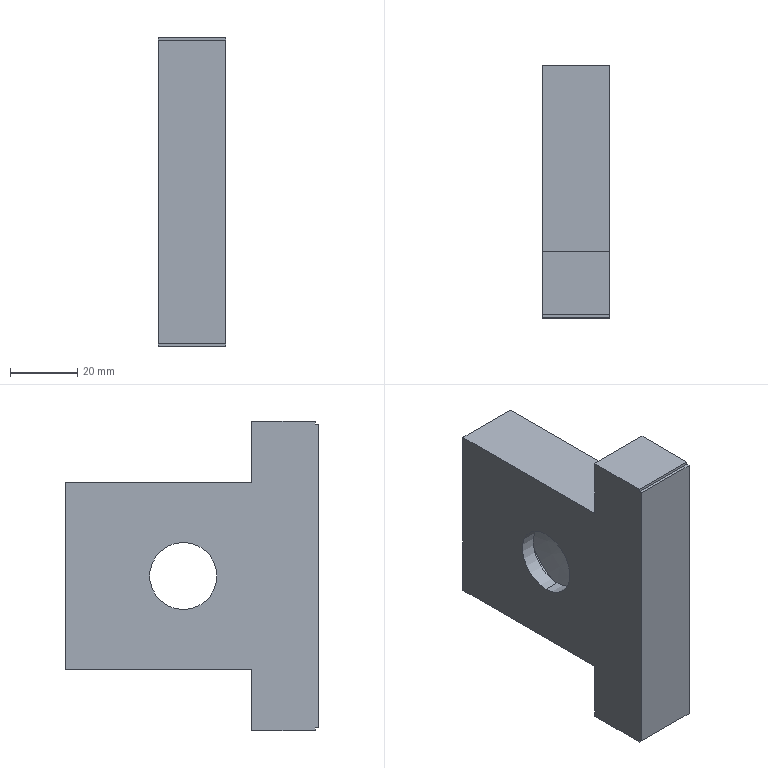Component | SolidWorks | SealingAnvil-1 | 1 solid | 24 faces | box 20 x 75.24 x 92.14 mm | volume 83671 mm3 | plane 14 | cylinder 6 | cone 4 | commonest cylinder face diameters 20 x4 41.575 x2
build123d program:
from build123d import *

# Parameters (mm, degrees)
SKETCH2_R           = 10
BOSS_EXTRUDE1_DEPTH = 20
SKETCH1_W           = 1.15
SKETCH1_H           = 1
CUT_EXTRUDE1_DEPTH  = 108.672


with BuildPart() as part:
    # Sketch2 → Boss-Extrude1 (new body)
    with BuildSketch(Plane.XY):
        Polygon((27.887, 95.24), (-27.887, 95.24), (-27.887, 39.822), (-46.072, 39.822), (-46.072, 20), (46.072, 20), (46.072, 39.822), (27.887, 39.822), align=None)
        with Locations((0, 60.219)):
            Circle(SKETCH2_R, mode=Mode.SUBTRACT)
    extrude(amount=BOSS_EXTRUDE1_DEPTH)

    # Sketch3 → Cut-Revolve1 (revolve, cut)
    with BuildSketch(Plane(origin=(0, 0, 0), x_dir=(0, 0, -1), z_dir=(1, 0, 0)), mode=Mode.PRIVATE) as cut_revolve1_sk:
        Polygon((-12.9, 81.007), (-15.408, 70.219), (-4.592, 70.219), (-7.1, 81.007), align=None)
    revolve(cut_revolve1_sk.sketch.rotate(Axis((0, 60.219, -248), (0, 0, 1)), 90), axis=Axis((0, 60.219, -248), (0, 0, 1)), mode=Mode.SUBTRACT)

    # Sketch1 → Cut-Extrude1 (cut, through all)
    with BuildSketch(Plane.XY.offset(20)):
        with Locations((-45.825, 20.4)):
            Rectangle(SKETCH1_W, SKETCH1_H)
        with Locations((45.825, 20.4)):
            Rectangle(SKETCH1_W, SKETCH1_H)
    extrude(amount=-CUT_EXTRUDE1_DEPTH, mode=Mode.SUBTRACT)


solid = part.part

# Placed as in the assembly
solid = solid.moved(Location((-166, 0, 0), (0, 90, 0)))
STEP:
#1=COLOUR_RGB('',0.7922,0.8196,0.9333);
#2=FILL_AREA_STYLE_COLOUR('',#1);
#3=FILL_AREA_STYLE('',(#2));
#4=SURFACE_STYLE_FILL_AREA(#3);
#5=SURFACE_SIDE_STYLE('',(#4));
#6=SURFACE_STYLE_USAGE(.BOTH.,#5);
#7=PRESENTATION_STYLE_ASSIGNMENT((#6));
#8=CARTESIAN_POINT('',(-6.028,2.371,-0.8184));
#9=VERTEX_POINT('',#8);
#10=CARTESIAN_POINT('',(-6.028,2.371,0.8184));
#11=VERTEX_POINT('',#10);
#12=CARTESIAN_POINT('',(-6.028,2.371,-0.));
#13=DIRECTION('',(-1.,0.,0.));
#14=DIRECTION('',(0.,0.,1.));
#15=AXIS2_PLACEMENT_3D('',#12,#13,#14);
#16=CIRCLE('',#15,0.8184);
#17=EDGE_CURVE('',#9,#11,#16,.T.);
#18=ORIENTED_EDGE('',*,*,#17,.F.);
#19=CARTESIAN_POINT('',(-6.256,2.371,-0.8184));
#20=VERTEX_POINT('',#19);
#21=CARTESIAN_POINT('',(-16.299,2.371,-0.8184));
#22=DIRECTION('',(-1.,0.,0.));
#23=VECTOR('',#22,39.37);
#24=LINE('',#21,#23);
#25=EDGE_CURVE('',#9,#20,#24,.T.);
#26=ORIENTED_EDGE('',*,*,#25,.T.);
#27=CARTESIAN_POINT('',(-6.256,2.371,0.8184));
#28=VERTEX_POINT('',#27);
#29=CARTESIAN_POINT('',(-6.256,2.371,-0.));
#30=DIRECTION('',(-1.,0.,0.));
#31=DIRECTION('',(0.,0.,1.));
#32=AXIS2_PLACEMENT_3D('',#29,#30,#31);
#33=CIRCLE('',#32,0.8184);
#34=EDGE_CURVE('',#20,#28,#33,.T.);
#35=ORIENTED_EDGE('',*,*,#34,.T.);
#36=CARTESIAN_POINT('',(-16.299,2.371,0.8184));
#37=DIRECTION('',(-1.,0.,0.));
#38=VECTOR('',#37,39.37);
#39=LINE('',#36,#38);
#40=EDGE_CURVE('',#11,#28,#39,.T.);
#41=ORIENTED_EDGE('',*,*,#40,.F.);
#42=EDGE_LOOP('',(#18,#26,#35,#41));
#43=FACE_OUTER_BOUND('',#42,.T.);
#44=CARTESIAN_POINT('',(-16.299,2.371,-0.));
#45=DIRECTION('',(-1.,0.,0.));
#46=DIRECTION('',(0.,0.,1.));
#47=AXIS2_PLACEMENT_3D('',#44,#45,#46);
#48=CYLINDRICAL_SURFACE('',#47,0.8184);
#49=ADVANCED_FACE('',(#43),#48,.F.);
#50=CARTESIAN_POINT('',(-6.355,2.371,-0.3937));
#51=VERTEX_POINT('',#50);
#52=CARTESIAN_POINT('',(-6.355,2.371,0.3937));
#53=VERTEX_POINT('',#52);
#54=CARTESIAN_POINT('',(-6.355,2.371,-0.));
#55=DIRECTION('',(-1.,0.,0.));
#56=DIRECTION('',(0.,0.,1.));
#57=AXIS2_PLACEMENT_3D('',#54,#55,#56);
#58=CIRCLE('',#57,0.3937);
#59=EDGE_CURVE('',#51,#53,#58,.T.);
#60=ORIENTED_EDGE('',*,*,#59,.T.);
#61=CARTESIAN_POINT('',(-6.355,2.371,0.3937));
#62=DIRECTION('',(0.2264,0.,0.974));
#63=VECTOR('',#62,39.37);
#64=LINE('',#61,#63);
#65=EDGE_CURVE('',#53,#28,#64,.T.);
#66=ORIENTED_EDGE('',*,*,#65,.T.);
#67=ORIENTED_EDGE('',*,*,#34,.F.);
#68=CARTESIAN_POINT('',(-6.355,2.371,-0.3937));
#69=DIRECTION('',(0.2264,0.,-0.974));
#70=VECTOR('',#69,39.37);
#71=LINE('',#68,#70);
#72=EDGE_CURVE('',#51,#20,#71,.T.);
#73=ORIENTED_EDGE('',*,*,#72,.F.);
#74=EDGE_LOOP('',(#60,#66,#67,#73));
#75=FACE_OUTER_BOUND('',#74,.T.);
#76=CARTESIAN_POINT('',(-6.355,2.371,-0.));
#77=DIRECTION('',(1.,0.,0.));
#78=DIRECTION('',(0.,0.,-1.));
#79=AXIS2_PLACEMENT_3D('',#76,#77,#78);
#80=CONICAL_SURFACE('',#79,0.3937,1.342);
#81=ADVANCED_FACE('',(#75),#80,.F.);
#82=CARTESIAN_POINT('',(-5.929,2.371,-0.3937));
#83=VERTEX_POINT('',#82);
#84=CARTESIAN_POINT('',(-5.929,2.371,0.3937));
#85=VERTEX_POINT('',#84);
#86=CARTESIAN_POINT('',(-5.929,2.371,-0.));
#87=DIRECTION('',(-1.,0.,0.));
#88=DIRECTION('',(0.,0.,1.));
#89=AXIS2_PLACEMENT_3D('',#86,#87,#88);
#90=CIRCLE('',#89,0.3937);
#91=EDGE_CURVE('',#83,#85,#90,.T.);
#92=ORIENTED_EDGE('',*,*,#91,.F.);
#93=CARTESIAN_POINT('',(-5.929,2.371,-0.3937));
#94=DIRECTION('',(-0.2264,0.,-0.974));
#95=VECTOR('',#94,39.37);
#96=LINE('',#93,#95);
#97=EDGE_CURVE('',#83,#9,#96,.T.);
#98=ORIENTED_EDGE('',*,*,#97,.T.);
#99=ORIENTED_EDGE('',*,*,#17,.T.);
#100=CARTESIAN_POINT('',(-5.929,2.371,0.3937));
#101=DIRECTION('',(-0.2264,0.,0.974));
#102=VECTOR('',#101,39.37);
#103=LINE('',#100,#102);
#104=EDGE_CURVE('',#85,#11,#103,.T.);
#105=ORIENTED_EDGE('',*,*,#104,.F.);
#106=EDGE_LOOP('',(#92,#98,#99,#105));
#107=FACE_OUTER_BOUND('',#106,.T.);
#108=CARTESIAN_POINT('',(-5.929,2.371,-0.));
#109=DIRECTION('',(-1.,0.,0.));
#110=DIRECTION('',(0.,0.,1.));
#111=AXIS2_PLACEMENT_3D('',#108,#109,#110);
#112=CONICAL_SURFACE('',#111,0.3937,1.342);
#113=ADVANCED_FACE('',(#107),#112,.F.);
#114=ORIENTED_EDGE('',*,*,#59,.F.);
#115=CARTESIAN_POINT('',(-6.535,2.371,-0.3937));
#116=VERTEX_POINT('',#115);
#117=CARTESIAN_POINT('',(-5.748,2.371,-0.3937));
#118=DIRECTION('',(-1.,0.,0.));
#119=VECTOR('',#118,39.37);
#120=LINE('',#117,#119);
#121=EDGE_CURVE('',#51,#116,#120,.T.);
#122=ORIENTED_EDGE('',*,*,#121,.T.);
#123=CARTESIAN_POINT('',(-6.535,2.371,0.3937));
#124=VERTEX_POINT('',#123);
#125=CARTESIAN_POINT('',(-6.535,2.371,-0.));
#126=DIRECTION('',(1.,0.,0.));
#127=DIRECTION('',(0.,0.,-1.));
#128=AXIS2_PLACEMENT_3D('',#125,#126,#127);
#129=CIRCLE('',#128,0.3937);
#130=EDGE_CURVE('',#124,#116,#129,.T.);
#131=ORIENTED_EDGE('',*,*,#130,.F.);
#132=CARTESIAN_POINT('',(-5.748,2.371,0.3937));
#133=DIRECTION('',(-1.,0.,0.));
#134=VECTOR('',#133,39.37);
#135=LINE('',#132,#134);
#136=EDGE_CURVE('',#53,#124,#135,.T.);
#137=ORIENTED_EDGE('',*,*,#136,.F.);
#138=EDGE_LOOP('',(#114,#122,#131,#137));
#139=FACE_OUTER_BOUND('',#138,.T.);
#140=CARTESIAN_POINT('',(-5.748,2.371,-0.));
#141=DIRECTION('',(-1.,0.,0.));
#142=DIRECTION('',(0.,0.,1.));
#143=AXIS2_PLACEMENT_3D('',#140,#141,#142);
#144=CYLINDRICAL_SURFACE('',#143,0.3937);
#145=ADVANCED_FACE('',(#139),#144,.F.);
#146=CARTESIAN_POINT('',(-5.748,2.371,0.3937));
#147=VERTEX_POINT('',#146);
#148=CARTESIAN_POINT('',(-5.748,2.371,-0.3937));
#149=VERTEX_POINT('',#148);
#150=CARTESIAN_POINT('',(-5.748,2.371,-0.));
#151=DIRECTION('',(1.,0.,0.));
#152=DIRECTION('',(0.,0.,-1.));
#153=AXIS2_PLACEMENT_3D('',#150,#151,#152);
#154=CIRCLE('',#153,0.3937);
#155=EDGE_CURVE('',#147,#149,#154,.T.);
#156=ORIENTED_EDGE('',*,*,#155,.T.);
#157=CARTESIAN_POINT('',(-5.748,2.371,-0.3937));
#158=DIRECTION('',(-1.,0.,0.));
#159=VECTOR('',#158,39.37);
#160=LINE('',#157,#159);
#161=EDGE_CURVE('',#149,#83,#160,.T.);
#162=ORIENTED_EDGE('',*,*,#161,.T.);
#163=ORIENTED_EDGE('',*,*,#91,.T.);
#164=CARTESIAN_POINT('',(-5.748,2.371,0.3937));
#165=DIRECTION('',(-1.,0.,0.));
#166=VECTOR('',#165,39.37);
#167=LINE('',#164,#166);
#168=EDGE_CURVE('',#147,#85,#167,.T.);
#169=ORIENTED_EDGE('',*,*,#168,.F.);
#170=EDGE_LOOP('',(#156,#162,#163,#169));
#171=FACE_OUTER_BOUND('',#170,.T.);
#172=CARTESIAN_POINT('',(-5.748,2.371,-0.));
#173=DIRECTION('',(-1.,0.,0.));
#174=DIRECTION('',(0.,0.,1.));
#175=AXIS2_PLACEMENT_3D('',#172,#173,#174);
#176=CYLINDRICAL_SURFACE('',#175,0.3937);
#177=ADVANCED_FACE('',(#171),#176,.F.);
#178=ORIENTED_EDGE('',*,*,#161,.F.);
#179=CARTESIAN_POINT('',(-5.748,2.371,-0.));
#180=DIRECTION('',(1.,0.,0.));
#181=DIRECTION('',(0.,0.,-1.));
#182=AXIS2_PLACEMENT_3D('',#179,#180,#181);
#183=CIRCLE('',#182,0.3937);
#184=EDGE_CURVE('',#149,#147,#183,.T.);
#185=ORIENTED_EDGE('',*,*,#184,.T.);
#186=ORIENTED_EDGE('',*,*,#168,.T.);
#187=CARTESIAN_POINT('',(-5.929,2.371,-0.));
#188=DIRECTION('',(-1.,0.,0.));
#189=DIRECTION('',(0.,0.,1.));
#190=AXIS2_PLACEMENT_3D('',#187,#188,#189);
#191=CIRCLE('',#190,0.3937);
#192=EDGE_CURVE('',#85,#83,#191,.T.);
#193=ORIENTED_EDGE('',*,*,#192,.T.);
#194=EDGE_LOOP('',(#178,#185,#186,#193));
#195=FACE_OUTER_BOUND('',#194,.T.);
#196=CARTESIAN_POINT('',(-5.748,2.371,-0.));
#197=DIRECTION('',(-1.,0.,0.));
#198=DIRECTION('',(0.,0.,1.));
#199=AXIS2_PLACEMENT_3D('',#196,#197,#198);
#200=CYLINDRICAL_SURFACE('',#199,0.3937);
#201=ADVANCED_FACE('',(#195),#200,.F.);
#202=CARTESIAN_POINT('',(-5.748,0.7874,1.781));
#203=VERTEX_POINT('',#202);
#204=CARTESIAN_POINT('',(-5.748,0.8228,1.781));
#205=VERTEX_POINT('',#204);
#206=CARTESIAN_POINT('',(-5.748,0.7835,1.781));
#207=DIRECTION('',(0.,1.,0.));
#208=VECTOR('',#207,39.37);
#209=LINE('',#206,#208);
#210=EDGE_CURVE('',#203,#205,#209,.T.);
#211=ORIENTED_EDGE('',*,*,#210,.F.);
#212=CARTESIAN_POINT('',(-5.748,0.7874,-1.781));
#213=VERTEX_POINT('',#212);
#214=CARTESIAN_POINT('',(-5.748,0.7874,1.814));
#215=DIRECTION('',(0.,0.,-1.));
#216=VECTOR('',#215,39.37);
#217=LINE('',#214,#216);
#218=EDGE_CURVE('',#203,#213,#217,.T.);
#219=ORIENTED_EDGE('',*,*,#218,.T.);
#220=CARTESIAN_POINT('',(-5.748,0.8228,-1.781));
#221=VERTEX_POINT('',#220);
#222=CARTESIAN_POINT('',(-5.748,0.7835,-1.781));
#223=DIRECTION('',(0.,-1.,0.));
#224=VECTOR('',#223,39.37);
#225=LINE('',#222,#224);
#226=EDGE_CURVE('',#221,#213,#225,.T.);
#227=ORIENTED_EDGE('',*,*,#226,.F.);
#228=CARTESIAN_POINT('',(-5.748,0.8228,-1.814));
#229=VERTEX_POINT('',#228);
#230=CARTESIAN_POINT('',(-5.748,0.8228,-1.827));
#231=DIRECTION('',(0.,0.,1.));
#232=VECTOR('',#231,39.37);
#233=LINE('',#230,#232);
#234=EDGE_CURVE('',#229,#221,#233,.T.);
#235=ORIENTED_EDGE('',*,*,#234,.F.);
#236=CARTESIAN_POINT('',(-5.748,1.568,-1.814));
#237=VERTEX_POINT('',#236);
#238=CARTESIAN_POINT('',(-5.748,0.7874,-1.814));
#239=DIRECTION('',(0.,1.,0.));
#240=VECTOR('',#239,39.37);
#241=LINE('',#238,#240);
#242=EDGE_CURVE('',#229,#237,#241,.T.);
#243=ORIENTED_EDGE('',*,*,#242,.T.);
#244=CARTESIAN_POINT('',(-5.748,1.568,-1.098));
#245=VERTEX_POINT('',#244);
#246=CARTESIAN_POINT('',(-5.748,1.568,-1.814));
#247=DIRECTION('',(0.,0.,1.));
#248=VECTOR('',#247,39.37);
#249=LINE('',#246,#248);
#250=EDGE_CURVE('',#237,#245,#249,.T.);
#251=ORIENTED_EDGE('',*,*,#250,.T.);
#252=CARTESIAN_POINT('',(-5.748,3.75,-1.098));
#253=VERTEX_POINT('',#252);
#254=CARTESIAN_POINT('',(-5.748,1.568,-1.098));
#255=DIRECTION('',(0.,1.,0.));
#256=VECTOR('',#255,39.37);
#257=LINE('',#254,#256);
#258=EDGE_CURVE('',#245,#253,#257,.T.);
#259=ORIENTED_EDGE('',*,*,#258,.T.);
#260=CARTESIAN_POINT('',(-5.748,3.75,1.098));
#261=VERTEX_POINT('',#260);
#262=CARTESIAN_POINT('',(-5.748,3.75,-1.098));
#263=DIRECTION('',(0.,0.,1.));
#264=VECTOR('',#263,39.37);
#265=LINE('',#262,#264);
#266=EDGE_CURVE('',#253,#261,#265,.T.);
#267=ORIENTED_EDGE('',*,*,#266,.T.);
#268=CARTESIAN_POINT('',(-5.748,1.568,1.098));
#269=VERTEX_POINT('',#268);
#270=CARTESIAN_POINT('',(-5.748,3.75,1.098));
#271=DIRECTION('',(0.,-1.,0.));
#272=VECTOR('',#271,39.37);
#273=LINE('',#270,#272);
#274=EDGE_CURVE('',#261,#269,#273,.T.);
#275=ORIENTED_EDGE('',*,*,#274,.T.);
#276=CARTESIAN_POINT('',(-5.748,1.568,1.814));
#277=VERTEX_POINT('',#276);
#278=CARTESIAN_POINT('',(-5.748,1.568,1.098));
#279=DIRECTION('',(0.,-0.,1.));
#280=VECTOR('',#279,39.37);
#281=LINE('',#278,#280);
#282=EDGE_CURVE('',#269,#277,#281,.T.);
#283=ORIENTED_EDGE('',*,*,#282,.T.);
#284=CARTESIAN_POINT('',(-5.748,0.8228,1.814));
#285=VERTEX_POINT('',#284);
#286=CARTESIAN_POINT('',(-5.748,1.568,1.814));
#287=DIRECTION('',(0.,-1.,-0.));
#288=VECTOR('',#287,39.37);
#289=LINE('',#286,#288);
#290=EDGE_CURVE('',#277,#285,#289,.T.);
#291=ORIENTED_EDGE('',*,*,#290,.T.);
#292=CARTESIAN_POINT('',(-5.748,0.8228,1.781));
#293=DIRECTION('',(0.,0.,1.));
#294=VECTOR('',#293,39.37);
#295=LINE('',#292,#294);
#296=EDGE_CURVE('',#205,#285,#295,.T.);
#297=ORIENTED_EDGE('',*,*,#296,.F.);
#298=EDGE_LOOP('',(#211,#219,#227,#235,#243,#251,#259,#267,#275,#283,#291,#297));
#299=FACE_OUTER_BOUND('',#298,.T.);
#300=ORIENTED_EDGE('',*,*,#155,.F.);
#301=ORIENTED_EDGE('',*,*,#184,.F.);
#302=EDGE_LOOP('',(#300,#301));
#303=FACE_BOUND('',#302,.T.);
#304=CARTESIAN_POINT('',(-5.748,-0.,-0.));
#305=DIRECTION('',(1.,0.,0.));
#306=DIRECTION('',(0.,0.,-1.));
#307=AXIS2_PLACEMENT_3D('',#304,#305,#306);
#308=PLANE('',#307);
#309=ADVANCED_FACE('',(#299,#303),#308,.T.);
#310=CARTESIAN_POINT('',(-6.535,0.7874,1.781));
#311=VERTEX_POINT('',#310);
#312=CARTESIAN_POINT('',(-6.535,0.7874,-1.781));
#313=VERTEX_POINT('',#312);
#314=CARTESIAN_POINT('',(-6.535,0.7874,1.814));
#315=DIRECTION('',(0.,0.,-1.));
#316=VECTOR('',#315,39.37);
#317=LINE('',#314,#316);
#318=EDGE_CURVE('',#311,#313,#317,.T.);
#319=ORIENTED_EDGE('',*,*,#318,.F.);
#320=CARTESIAN_POINT('',(-6.535,0.8228,1.781));
#321=VERTEX_POINT('',#320);
#322=CARTESIAN_POINT('',(-6.535,0.7835,1.781));
#323=DIRECTION('',(0.,1.,0.));
#324=VECTOR('',#323,39.37);
#325=LINE('',#322,#324);
#326=EDGE_CURVE('',#311,#321,#325,.T.);
#327=ORIENTED_EDGE('',*,*,#326,.T.);
#328=CARTESIAN_POINT('',(-6.535,0.8228,1.814));
#329=VERTEX_POINT('',#328);
#330=CARTESIAN_POINT('',(-6.535,0.8228,1.781));
#331=DIRECTION('',(0.,0.,1.));
#332=VECTOR('',#331,39.37);
#333=LINE('',#330,#332);
#334=EDGE_CURVE('',#321,#329,#333,.T.);
#335=ORIENTED_EDGE('',*,*,#334,.T.);
#336=CARTESIAN_POINT('',(-6.535,1.568,1.814));
#337=VERTEX_POINT('',#336);
#338=CARTESIAN_POINT('',(-6.535,1.568,1.814));
#339=DIRECTION('',(0.,-1.,-0.));
#340=VECTOR('',#339,39.37);
#341=LINE('',#338,#340);
#342=EDGE_CURVE('',#337,#329,#341,.T.);
#343=ORIENTED_EDGE('',*,*,#342,.F.);
#344=CARTESIAN_POINT('',(-6.535,1.568,1.098));
#345=VERTEX_POINT('',#344);
#346=CARTESIAN_POINT('',(-6.535,1.568,1.098));
#347=DIRECTION('',(0.,-0.,1.));
#348=VECTOR('',#347,39.37);
#349=LINE('',#346,#348);
#350=EDGE_CURVE('',#345,#337,#349,.T.);
#351=ORIENTED_EDGE('',*,*,#350,.F.);
#352=CARTESIAN_POINT('',(-6.535,3.75,1.098));
#353=VERTEX_POINT('',#352);
#354=CARTESIAN_POINT('',(-6.535,3.75,1.098));
#355=DIRECTION('',(0.,-1.,0.));
#356=VECTOR('',#355,39.37);
#357=LINE('',#354,#356);
#358=EDGE_CURVE('',#353,#345,#357,.T.);
#359=ORIENTED_EDGE('',*,*,#358,.F.);
#360=CARTESIAN_POINT('',(-6.535,3.75,-1.098));
#361=VERTEX_POINT('',#360);
#362=CARTESIAN_POINT('',(-6.535,3.75,-1.098));
#363=DIRECTION('',(0.,0.,1.));
#364=VECTOR('',#363,39.37);
#365=LINE('',#362,#364);
#366=EDGE_CURVE('',#361,#353,#365,.T.);
#367=ORIENTED_EDGE('',*,*,#366,.F.);
#368=CARTESIAN_POINT('',(-6.535,1.568,-1.098));
#369=VERTEX_POINT('',#368);
#370=CARTESIAN_POINT('',(-6.535,1.568,-1.098));
#371=DIRECTION('',(0.,1.,0.));
#372=VECTOR('',#371,39.37);
#373=LINE('',#370,#372);
#374=EDGE_CURVE('',#369,#361,#373,.T.);
#375=ORIENTED_EDGE('',*,*,#374,.F.);
#376=CARTESIAN_POINT('',(-6.535,1.568,-1.814));
#377=VERTEX_POINT('',#376);
#378=CARTESIAN_POINT('',(-6.535,1.568,-1.814));
#379=DIRECTION('',(0.,0.,1.));
#380=VECTOR('',#379,39.37);
#381=LINE('',#378,#380);
#382=EDGE_CURVE('',#377,#369,#381,.T.);
#383=ORIENTED_EDGE('',*,*,#382,.F.);
#384=CARTESIAN_POINT('',(-6.535,0.8228,-1.814));
#385=VERTEX_POINT('',#384);
#386=CARTESIAN_POINT('',(-6.535,0.7874,-1.814));
#387=DIRECTION('',(0.,1.,0.));
#388=VECTOR('',#387,39.37);
#389=LINE('',#386,#388);
#390=EDGE_CURVE('',#385,#377,#389,.T.);
#391=ORIENTED_EDGE('',*,*,#390,.F.);
#392=CARTESIAN_POINT('',(-6.535,0.8228,-1.781));
#393=VERTEX_POINT('',#392);
#394=CARTESIAN_POINT('',(-6.535,0.8228,-1.827));
#395=DIRECTION('',(0.,0.,1.));
#396=VECTOR('',#395,39.37);
#397=LINE('',#394,#396);
#398=EDGE_CURVE('',#385,#393,#397,.T.);
#399=ORIENTED_EDGE('',*,*,#398,.T.);
#400=CARTESIAN_POINT('',(-6.535,0.7835,-1.781));
#401=DIRECTION('',(0.,-1.,0.));
#402=VECTOR('',#401,39.37);
#403=LINE('',#400,#402);
#404=EDGE_CURVE('',#393,#313,#403,.T.);
#405=ORIENTED_EDGE('',*,*,#404,.T.);
#406=EDGE_LOOP('',(#319,#327,#335,#343,#351,#359,#367,#375,#383,#391,#399,#405));
#407=FACE_OUTER_BOUND('',#406,.T.);
#408=ORIENTED_EDGE('',*,*,#130,.T.);
#409=CARTESIAN_POINT('',(-6.535,2.371,-0.));
#410=DIRECTION('',(1.,0.,0.));
#411=DIRECTION('',(0.,0.,-1.));
#412=AXIS2_PLACEMENT_3D('',#409,#410,#411);
#413=CIRCLE('',#412,0.3937);
#414=EDGE_CURVE('',#116,#124,#413,.T.);
#415=ORIENTED_EDGE('',*,*,#414,.T.);
#416=EDGE_LOOP('',(#408,#415));
#417=FACE_BOUND('',#416,.T.);
#418=CARTESIAN_POINT('',(-6.535,-0.,-0.));
#419=DIRECTION('',(1.,0.,0.));
#420=DIRECTION('',(0.,0.,-1.));
#421=AXIS2_PLACEMENT_3D('',#418,#419,#420);
#422=PLANE('',#421);
#423=ADVANCED_FACE('',(#407,#417),#422,.F.);
#424=ORIENTED_EDGE('',*,*,#374,.T.);
#425=CARTESIAN_POINT('',(-5.748,3.75,-1.098));
#426=DIRECTION('',(-1.,0.,0.));
#427=VECTOR('',#426,39.37);
#428=LINE('',#425,#427);
#429=EDGE_CURVE('',#253,#361,#428,.T.);
#430=ORIENTED_EDGE('',*,*,#429,.F.);
#431=ORIENTED_EDGE('',*,*,#258,.F.);
#432=CARTESIAN_POINT('',(-5.748,1.568,-1.098));
#433=DIRECTION('',(-1.,0.,0.));
#434=VECTOR('',#433,39.37);
#435=LINE('',#432,#434);
#436=EDGE_CURVE('',#245,#369,#435,.T.);
#437=ORIENTED_EDGE('',*,*,#436,.T.);
#438=EDGE_LOOP('',(#424,#430,#431,#437));
#439=FACE_OUTER_BOUND('',#438,.T.);
#440=CARTESIAN_POINT('',(-5.748,1.568,-1.098));
#441=DIRECTION('',(0.,0.,1.));
#442=DIRECTION('',(1.,0.,0.));
#443=AXIS2_PLACEMENT_3D('',#440,#441,#442);
#444=PLANE('',#443);
#445=ADVANCED_FACE('',(#439),#444,.F.);
#446=ORIENTED_EDGE('',*,*,#366,.T.);
#447=CARTESIAN_POINT('',(-5.748,3.75,1.098));
#448=DIRECTION('',(-1.,0.,0.));
#449=VECTOR('',#448,39.37);
#450=LINE('',#447,#449);
#451=EDGE_CURVE('',#261,#353,#450,.T.);
#452=ORIENTED_EDGE('',*,*,#451,.F.);
#453=ORIENTED_EDGE('',*,*,#266,.F.);
#454=ORIENTED_EDGE('',*,*,#429,.T.);
#455=EDGE_LOOP('',(#446,#452,#453,#454));
#456=FACE_OUTER_BOUND('',#455,.T.);
#457=CARTESIAN_POINT('',(-5.748,3.75,-1.098));
#458=DIRECTION('',(0.,-1.,0.));
#459=DIRECTION('',(-1.,0.,0.));
#460=AXIS2_PLACEMENT_3D('',#457,#458,#459);
#461=PLANE('',#460);
#462=ADVANCED_FACE('',(#456),#461,.F.);
#463=ORIENTED_EDGE('',*,*,#358,.T.);
#464=CARTESIAN_POINT('',(-5.748,1.568,1.098));
#465=DIRECTION('',(-1.,0.,0.));
#466=VECTOR('',#465,39.37);
#467=LINE('',#464,#466);
#468=EDGE_CURVE('',#269,#345,#467,.T.);
#469=ORIENTED_EDGE('',*,*,#468,.F.);
#470=ORIENTED_EDGE('',*,*,#274,.F.);
#471=ORIENTED_EDGE('',*,*,#451,.T.);
#472=EDGE_LOOP('',(#463,#469,#470,#471));
#473=FACE_OUTER_BOUND('',#472,.T.);
#474=CARTESIAN_POINT('',(-5.748,3.75,1.098));
#475=DIRECTION('',(0.,0.,-1.));
#476=DIRECTION('',(-1.,0.,0.));
#477=AXIS2_PLACEMENT_3D('',#474,#475,#476);
#478=PLANE('',#477);
#479=ADVANCED_FACE('',(#473),#478,.F.);
#480=ORIENTED_EDGE('',*,*,#350,.T.);
#481=CARTESIAN_POINT('',(-5.748,1.568,1.814));
#482=DIRECTION('',(-1.,0.,0.));
#483=VECTOR('',#482,39.37);
#484=LINE('',#481,#483);
#485=EDGE_CURVE('',#277,#337,#484,.T.);
#486=ORIENTED_EDGE('',*,*,#485,.F.);
#487=ORIENTED_EDGE('',*,*,#282,.F.);
#488=ORIENTED_EDGE('',*,*,#468,.T.);
#489=EDGE_LOOP('',(#480,#486,#487,#488));
#490=FACE_OUTER_BOUND('',#489,.T.);
#491=CARTESIAN_POINT('',(-5.748,1.568,1.098));
#492=DIRECTION('',(0.,-1.,-0.));
#493=DIRECTION('',(0.,0.,-1.));
#494=AXIS2_PLACEMENT_3D('',#491,#492,#493);
#495=PLANE('',#494);
#496=ADVANCED_FACE('',(#490),#495,.F.);
#497=ORIENTED_EDGE('',*,*,#342,.T.);
#498=CARTESIAN_POINT('',(-5.748,0.8228,1.814));
#499=DIRECTION('',(1.,0.,0.));
#500=VECTOR('',#499,39.37);
#501=LINE('',#498,#500);
#502=EDGE_CURVE('',#329,#285,#501,.T.);
#503=ORIENTED_EDGE('',*,*,#502,.T.);
#504=ORIENTED_EDGE('',*,*,#290,.F.);
#505=ORIENTED_EDGE('',*,*,#485,.T.);
#506=EDGE_LOOP('',(#497,#503,#504,#505));
#507=FACE_OUTER_BOUND('',#506,.T.);
#508=CARTESIAN_POINT('',(-5.748,1.568,1.814));
#509=DIRECTION('',(0.,0.,-1.));
#510=DIRECTION('',(0.,1.,0.));
#511=AXIS2_PLACEMENT_3D('',#508,#509,#510);
#512=PLANE('',#511);
#513=ADVANCED_FACE('',(#507),#512,.F.);
#514=ORIENTED_EDGE('',*,*,#218,.F.);
#515=CARTESIAN_POINT('',(-5.748,0.7874,1.781));
#516=DIRECTION('',(-1.,0.,0.));
#517=VECTOR('',#516,39.37);
#518=LINE('',#515,#517);
#519=EDGE_CURVE('',#203,#311,#518,.T.);
#520=ORIENTED_EDGE('',*,*,#519,.T.);
#521=ORIENTED_EDGE('',*,*,#318,.T.);
#522=CARTESIAN_POINT('',(-5.748,0.7874,-1.781));
#523=DIRECTION('',(1.,0.,0.));
#524=VECTOR('',#523,39.37);
#525=LINE('',#522,#524);
#526=EDGE_CURVE('',#313,#213,#525,.T.);
#527=ORIENTED_EDGE('',*,*,#526,.T.);
#528=EDGE_LOOP('',(#514,#520,#521,#527));
#529=FACE_OUTER_BOUND('',#528,.T.);
#530=CARTESIAN_POINT('',(-5.748,0.7874,1.814));
#531=DIRECTION('',(0.,1.,0.));
#532=DIRECTION('',(0.,-0.,1.));
#533=AXIS2_PLACEMENT_3D('',#530,#531,#532);
#534=PLANE('',#533);
#535=ADVANCED_FACE('',(#529),#534,.F.);
#536=ORIENTED_EDGE('',*,*,#242,.F.);
#537=CARTESIAN_POINT('',(-5.748,0.8228,-1.814));
#538=DIRECTION('',(-1.,0.,0.));
#539=VECTOR('',#538,39.37);
#540=LINE('',#537,#539);
#541=EDGE_CURVE('',#229,#385,#540,.T.);
#542=ORIENTED_EDGE('',*,*,#541,.T.);
#543=ORIENTED_EDGE('',*,*,#390,.T.);
#544=CARTESIAN_POINT('',(-5.748,1.568,-1.814));
#545=DIRECTION('',(-1.,0.,0.));
#546=VECTOR('',#545,39.37);
#547=LINE('',#544,#546);
#548=EDGE_CURVE('',#237,#377,#547,.T.);
#549=ORIENTED_EDGE('',*,*,#548,.F.);
#550=EDGE_LOOP('',(#536,#542,#543,#549));
#551=FACE_OUTER_BOUND('',#550,.T.);
#552=CARTESIAN_POINT('',(-5.748,0.7874,-1.814));
#553=DIRECTION('',(0.,0.,1.));
#554=DIRECTION('',(1.,0.,0.));
#555=AXIS2_PLACEMENT_3D('',#552,#553,#554);
#556=PLANE('',#555);
#557=ADVANCED_FACE('',(#551),#556,.F.);
#558=ORIENTED_EDGE('',*,*,#382,.T.);
#559=ORIENTED_EDGE('',*,*,#436,.F.);
#560=ORIENTED_EDGE('',*,*,#250,.F.);
#561=ORIENTED_EDGE('',*,*,#548,.T.);
#562=EDGE_LOOP('',(#558,#559,#560,#561));
#563=FACE_OUTER_BOUND('',#562,.T.);
#564=CARTESIAN_POINT('',(-5.748,1.568,-1.814));
#565=DIRECTION('',(0.,-1.,0.));
#566=DIRECTION('',(-1.,0.,0.));
#567=AXIS2_PLACEMENT_3D('',#564,#565,#566);
#568=PLANE('',#567);
#569=ADVANCED_FACE('',(#563),#568,.F.);
#570=ORIENTED_EDGE('',*,*,#121,.F.);
#571=CARTESIAN_POINT('',(-6.355,2.371,-0.));
#572=DIRECTION('',(-1.,0.,0.));
#573=DIRECTION('',(0.,0.,1.));
#574=AXIS2_PLACEMENT_3D('',#571,#572,#573);
#575=CIRCLE('',#574,0.3937);
#576=EDGE_CURVE('',#53,#51,#575,.T.);
#577=ORIENTED_EDGE('',*,*,#576,.F.);
#578=ORIENTED_EDGE('',*,*,#136,.T.);
#579=ORIENTED_EDGE('',*,*,#414,.F.);
#580=EDGE_LOOP('',(#570,#577,#578,#579));
#581=FACE_OUTER_BOUND('',#580,.T.);
#582=CARTESIAN_POINT('',(-5.748,2.371,-0.));
#583=DIRECTION('',(-1.,0.,0.));
#584=DIRECTION('',(0.,0.,1.));
#585=AXIS2_PLACEMENT_3D('',#582,#583,#584);
#586=CYLINDRICAL_SURFACE('',#585,0.3937);
#587=ADVANCED_FACE('',(#581),#586,.F.);
#588=ORIENTED_EDGE('',*,*,#97,.F.);
#589=ORIENTED_EDGE('',*,*,#192,.F.);
#590=ORIENTED_EDGE('',*,*,#104,.T.);
#591=CARTESIAN_POINT('',(-6.028,2.371,-0.));
#592=DIRECTION('',(-1.,0.,0.));
#593=DIRECTION('',(0.,0.,1.));
#594=AXIS2_PLACEMENT_3D('',#591,#592,#593);
#595=CIRCLE('',#594,0.8184);
#596=EDGE_CURVE('',#11,#9,#595,.T.);
#597=ORIENTED_EDGE('',*,*,#596,.T.);
#598=EDGE_LOOP('',(#588,#589,#590,#597));
#599=FACE_OUTER_BOUND('',#598,.T.);
#600=CARTESIAN_POINT('',(-5.929,2.371,-0.));
#601=DIRECTION('',(-1.,0.,0.));
#602=DIRECTION('',(0.,0.,1.));
#603=AXIS2_PLACEMENT_3D('',#600,#601,#602);
#604=CONICAL_SURFACE('',#603,0.3937,1.342);
#605=ADVANCED_FACE('',(#599),#604,.F.);
#606=ORIENTED_EDGE('',*,*,#65,.F.);
#607=ORIENTED_EDGE('',*,*,#576,.T.);
#608=ORIENTED_EDGE('',*,*,#72,.T.);
#609=CARTESIAN_POINT('',(-6.256,2.371,-0.));
#610=DIRECTION('',(-1.,0.,0.));
#611=DIRECTION('',(0.,0.,1.));
#612=AXIS2_PLACEMENT_3D('',#609,#610,#611);
#613=CIRCLE('',#612,0.8184);
#614=EDGE_CURVE('',#28,#20,#613,.T.);
#615=ORIENTED_EDGE('',*,*,#614,.F.);
#616=EDGE_LOOP('',(#606,#607,#608,#615));
#617=FACE_OUTER_BOUND('',#616,.T.);
#618=CARTESIAN_POINT('',(-6.355,2.371,-0.));
#619=DIRECTION('',(1.,0.,0.));
#620=DIRECTION('',(0.,0.,-1.));
#621=AXIS2_PLACEMENT_3D('',#618,#619,#620);
#622=CONICAL_SURFACE('',#621,0.3937,1.342);
#623=ADVANCED_FACE('',(#617),#622,.F.);
#624=ORIENTED_EDGE('',*,*,#25,.F.);
#625=ORIENTED_EDGE('',*,*,#596,.F.);
#626=ORIENTED_EDGE('',*,*,#40,.T.);
#627=ORIENTED_EDGE('',*,*,#614,.T.);
#628=EDGE_LOOP('',(#624,#625,#626,#627));
#629=FACE_OUTER_BOUND('',#628,.T.);
#630=CARTESIAN_POINT('',(-16.299,2.371,-0.));
#631=DIRECTION('',(-1.,0.,0.));
#632=DIRECTION('',(0.,0.,1.));
#633=AXIS2_PLACEMENT_3D('',#630,#631,#632);
#634=CYLINDRICAL_SURFACE('',#633,0.8184);
#635=ADVANCED_FACE('',(#629),#634,.F.);
#636=ORIENTED_EDGE('',*,*,#404,.F.);
#637=CARTESIAN_POINT('',(-6.535,0.8228,-1.781));
#638=DIRECTION('',(1.,0.,0.));
#639=VECTOR('',#638,39.37);
#640=LINE('',#637,#639);
#641=EDGE_CURVE('',#393,#221,#640,.T.);
#642=ORIENTED_EDGE('',*,*,#641,.T.);
#643=ORIENTED_EDGE('',*,*,#226,.T.);
#644=ORIENTED_EDGE('',*,*,#526,.F.);
#645=EDGE_LOOP('',(#636,#642,#643,#644));
#646=FACE_OUTER_BOUND('',#645,.T.);
#647=CARTESIAN_POINT('',(-6.535,0.7835,-1.781));
#648=DIRECTION('',(0.,0.,1.));
#649=DIRECTION('',(1.,0.,0.));
#650=AXIS2_PLACEMENT_3D('',#647,#648,#649);
#651=PLANE('',#650);
#652=ADVANCED_FACE('',(#646),#651,.F.);
#653=ORIENTED_EDGE('',*,*,#234,.T.);
#654=ORIENTED_EDGE('',*,*,#641,.F.);
#655=ORIENTED_EDGE('',*,*,#398,.F.);
#656=ORIENTED_EDGE('',*,*,#541,.F.);
#657=EDGE_LOOP('',(#653,#654,#655,#656));
#658=FACE_OUTER_BOUND('',#657,.T.);
#659=CARTESIAN_POINT('',(-6.535,0.8228,-1.827));
#660=DIRECTION('',(0.,1.,0.));
#661=DIRECTION('',(1.,0.,0.));
#662=AXIS2_PLACEMENT_3D('',#659,#660,#661);
#663=PLANE('',#662);
#664=ADVANCED_FACE('',(#658),#663,.F.);
#665=ORIENTED_EDGE('',*,*,#334,.F.);
#666=CARTESIAN_POINT('',(-6.535,0.8228,1.781));
#667=DIRECTION('',(1.,0.,0.));
#668=VECTOR('',#667,39.37);
#669=LINE('',#666,#668);
#670=EDGE_CURVE('',#321,#205,#669,.T.);
#671=ORIENTED_EDGE('',*,*,#670,.T.);
#672=ORIENTED_EDGE('',*,*,#296,.T.);
#673=ORIENTED_EDGE('',*,*,#502,.F.);
#674=EDGE_LOOP('',(#665,#671,#672,#673));
#675=FACE_OUTER_BOUND('',#674,.T.);
#676=CARTESIAN_POINT('',(-6.535,0.8228,1.781));
#677=DIRECTION('',(0.,1.,0.));
#678=DIRECTION('',(1.,0.,0.));
#679=AXIS2_PLACEMENT_3D('',#676,#677,#678);
#680=PLANE('',#679);
#681=ADVANCED_FACE('',(#675),#680,.F.);
#682=ORIENTED_EDGE('',*,*,#210,.T.);
#683=ORIENTED_EDGE('',*,*,#670,.F.);
#684=ORIENTED_EDGE('',*,*,#326,.F.);
#685=ORIENTED_EDGE('',*,*,#519,.F.);
#686=EDGE_LOOP('',(#682,#683,#684,#685));
#687=FACE_OUTER_BOUND('',#686,.T.);
#688=CARTESIAN_POINT('',(-6.535,0.7835,1.781));
#689=DIRECTION('',(0.,0.,-1.));
#690=DIRECTION('',(-1.,0.,0.));
#691=AXIS2_PLACEMENT_3D('',#688,#689,#690);
#692=PLANE('',#691);
#693=ADVANCED_FACE('',(#687),#692,.F.);
#694=CLOSED_SHELL('',(#49,#81,#113,#145,#177,#201,#309,#423,#445,#462,#479,#496,#513,#535,#557,#569,#587,#605,#623,#635,#652,#664,#681,#693));
#695=MANIFOLD_SOLID_BREP('',#694);
#696=STYLED_ITEM('',(#7),#695);
#697=PRESENTATION_LAYER_ASSIGNMENT('','',(#696));
#698=CARTESIAN_POINT('',(0.,0.,0.));
#699=DIRECTION('',(0.,0.,1.));
#700=DIRECTION('',(1.,0.,0.));
#701=AXIS2_PLACEMENT_3D('',#698,#699,#700);
#702=(LENGTH_UNIT()NAMED_UNIT(*)SI_UNIT($,.METRE.));
#703=LENGTH_MEASURE_WITH_UNIT(LENGTH_MEASURE(0.0254),#702);
#704=DIMENSIONAL_EXPONENTS(1.,0.,0.,0.,0.,0.,0.);
#705=(CONVERSION_BASED_UNIT('',#703)LENGTH_UNIT()NAMED_UNIT(#704));
#706=UNCERTAINTY_MEASURE_WITH_UNIT(LENGTH_MEASURE(0.00001),#705,'','');
#707=(NAMED_UNIT(*)PLANE_ANGLE_UNIT()SI_UNIT($,.RADIAN.));
#708=(NAMED_UNIT(*)SI_UNIT($,.STERADIAN.)SOLID_ANGLE_UNIT());
#709=(GEOMETRIC_REPRESENTATION_CONTEXT(3)GLOBAL_UNCERTAINTY_ASSIGNED_CONTEXT((#706))GLOBAL_UNIT_ASSIGNED_CONTEXT((#705,#707,#708))REPRESENTATION_CONTEXT('',''));
#710=ADVANCED_BREP_SHAPE_REPRESENTATION('',(#695,#701),#709);
#711=(LENGTH_UNIT()NAMED_UNIT(*)SI_UNIT($,.METRE.));
#712=LENGTH_MEASURE_WITH_UNIT(LENGTH_MEASURE(0.0254),#711);
#713=DIMENSIONAL_EXPONENTS(1.,0.,0.,0.,0.,0.,0.);
#714=(CONVERSION_BASED_UNIT('',#712)LENGTH_UNIT()NAMED_UNIT(#713));
#715=UNCERTAINTY_MEASURE_WITH_UNIT(LENGTH_MEASURE(0.00001),#714,'','');
#716=(NAMED_UNIT(*)PLANE_ANGLE_UNIT()SI_UNIT($,.RADIAN.));
#717=(NAMED_UNIT(*)SI_UNIT($,.STERADIAN.)SOLID_ANGLE_UNIT());
#718=(GEOMETRIC_REPRESENTATION_CONTEXT(3)GLOBAL_UNCERTAINTY_ASSIGNED_CONTEXT((#715))GLOBAL_UNIT_ASSIGNED_CONTEXT((#714,#716,#717))REPRESENTATION_CONTEXT('',''));
#719=MECHANICAL_DESIGN_GEOMETRIC_PRESENTATION_REPRESENTATION('',(#696),#718);